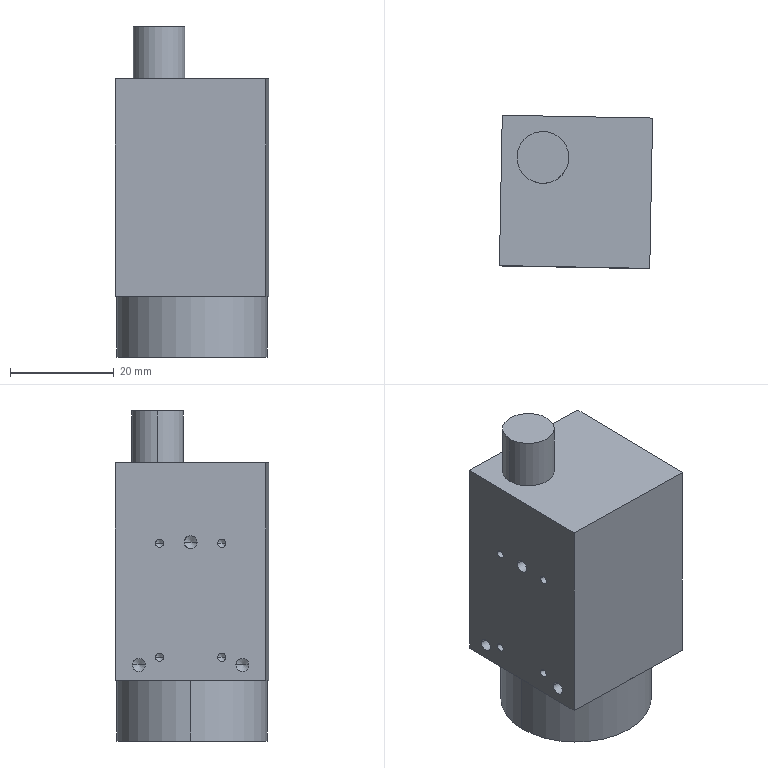Component | SolidWorks | HikvisionCamera-MV-CA060-10GM-2 | 1 solid | 55 faces | box 29.54 x 29.54 x 63.68 mm | volume 37314 mm3 | cylinder 24 | plane 17 | cone 14 | commonest cylinder face diameters 1.6 x8 2.5 x6 2 x4 10 x2 26 x2 29 x2 | material S45C
build123d program:
from build123d import *

# Parameters (mm, degrees)
SKETCH1_W             = 29
SKETCH1_H             = 29
BOSS_EXTRUDE1_DEPTH   = 42
SKETCH2_R             = 14.5
SKETCH2_R_2           = 13
BOSS_EXTRUDE2_DEPTH   = 11.679
M3_TAPPED_HOLE1_D     = 2.5
M3_TAPPED_HOLE1_DEPTH = 3
M3_TAPPED_HOLE1_TIP   = 0.7511
M2_TAPPED_HOLE1_D     = 1.6
M2_TAPPED_HOLE1_DEPTH = 3
M2_TAPPED_HOLE1_TIP   = 0.4807
SKETCH5_R             = 5
BOSS_EXTRUDE3_DEPTH   = 10
SKETCH6_W             = 18
SKETCH6_H             = 13
CUT_EXTRUDE1_DEPTH    = 1
FILLET1_R             = 1


with BuildPart() as part:
    # Sketch1 → Boss-Extrude1 (new body)
    with BuildSketch(Plane(origin=(0, 0, 0), x_dir=(1, 0, 0), z_dir=(0, 1, 0))):
        Rectangle(SKETCH1_W, SKETCH1_H)
    extrude(amount=BOSS_EXTRUDE1_DEPTH)

    # Sketch2 → Boss-Extrude2 (add)
    with BuildSketch(Plane.XZ):
        with Locations(Location((0, 0, 0), (0, 0, 270))):
            Circle(SKETCH2_R)
        with Locations(Location((0, 0, 0), (0, 0, 270))):
            Circle(SKETCH2_R_2, mode=Mode.SUBTRACT)
    extrude(amount=BOSS_EXTRUDE2_DEPTH)

    # M3 Tapped Hole1
    with Locations(Plane(origin=(-10, 3, 14.5), x_dir=(1, 0, 0), z_dir=(0, 0, 1))):
        with Locations((0, 0), (20, 0), (10, 23.7)):
            Hole(M3_TAPPED_HOLE1_D / 2, depth=M3_TAPPED_HOLE1_DEPTH)
            with Locations((0, 0, -(M3_TAPPED_HOLE1_DEPTH + M3_TAPPED_HOLE1_TIP / 2))):  # 118° drill point
                Cone(0, M3_TAPPED_HOLE1_D / 2, M3_TAPPED_HOLE1_TIP, mode=Mode.SUBTRACT)

    # M2 Tapped Hole1
    with Locations(Plane(origin=(-6, 4.5, 14.5), x_dir=(1, 0, 0), z_dir=(0, 0, 1))):
        with Locations((0, 0), (12, 0), (12, 22), (0, 22)):
            Hole(M2_TAPPED_HOLE1_D / 2, depth=M2_TAPPED_HOLE1_DEPTH)
            with Locations((0, 0, -(M2_TAPPED_HOLE1_DEPTH + M2_TAPPED_HOLE1_TIP / 2))):  # 118° drill point
                Cone(0, M2_TAPPED_HOLE1_D / 2, M2_TAPPED_HOLE1_TIP, mode=Mode.SUBTRACT)

    # Sketch5 → Boss-Extrude3 (add)
    with BuildSketch(Plane(origin=(0, 42, 0), x_dir=(1, 0, 0), z_dir=(0, 1, 0))):
        with Locations(Location((-6.5, -6.5, 0), (0, 0, 90))):
            Circle(SKETCH5_R)
    extrude(amount=BOSS_EXTRUDE3_DEPTH)

    # Sketch6 → Cut-Extrude1 (cut)
    with BuildSketch(Plane.XZ):
        Rectangle(SKETCH6_W, SKETCH6_H)
    extrude(amount=-CUT_EXTRUDE1_DEPTH, mode=Mode.SUBTRACT)

    # Fillet1
    fillet1_edges = [part.edges().sort_by_distance(p)[0] for p in [
        (-9, 0.5, -6.5),
        (-9, 0.5, 6.5),
        (9, 0.5, 6.5),
        (9, 0.5, -6.5),
    ]]
    fillet(fillet1_edges, radius=FILLET1_R)


solid = part.part

# Placed as in the assembly
solid = solid.moved(Location((541.864, 441.164, 1027.565), (-90, -88.927, -180)))